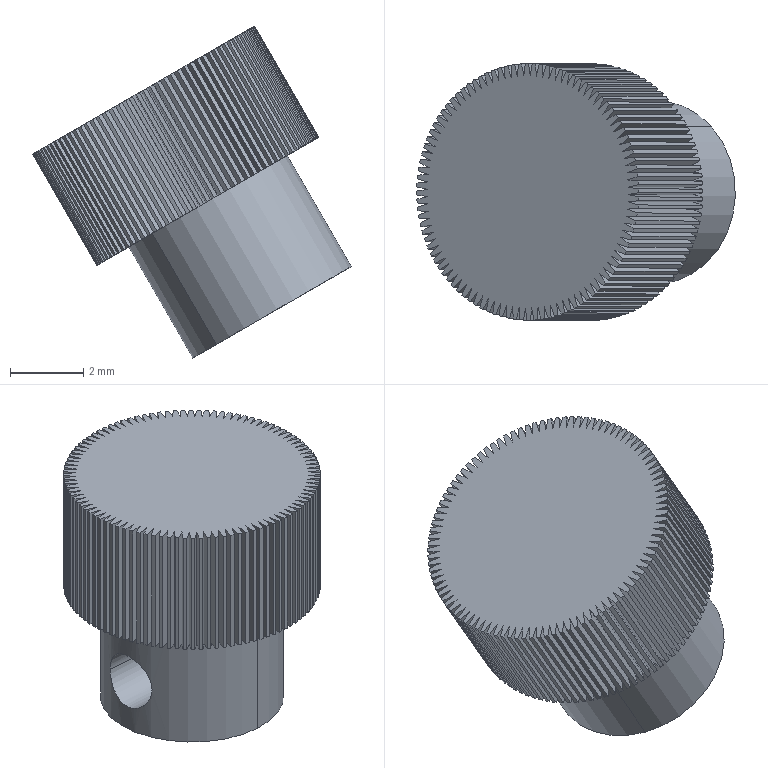Component | SolidWorks | SliderNut2-2 | 1 solid | 310 faces | box 8.7 x 7 x 9.06 mm | volume 183 mm3 | plane 204 | cylinder 106 | commonest cylinder face diameters 7 x100 1.6 x2 2 x2 5 x2
build123d program:
from build123d import *

# Parameters (mm, degrees)
SKETCH2_R               = 1
CUT_EXTRUDE1_DEPTH      = 3.5
CUT_EXTRUDE2_REACH      = 9.778
CUT_EXTRUDE2_END_RADIUS = 1
SKETCH3_R               = 0.8
CUT_EXTRUDE3_DEPTH      = 3.5


with BuildPart() as part:
    # Sketch1 → Revolve1 (revolve)
    with BuildSketch(Plane.XY, mode=Mode.PRIVATE) as revolve1_sk:
        Polygon((-3.5, 0), (3.5, 0), (3.5, 2.5), (0, 2.5), (0, 3.5), (-3.5, 3.5), align=None)
    revolve(revolve1_sk.sketch.rotate(Axis((-3.5, 0, 0), (1, 0, 0)), 90), axis=Axis((-3.5, 0, 0), (1, 0, 0)))

    # Sketch2 → Cut-Extrude1 (cut)
    with BuildSketch(Plane(origin=(3.5, 0, 0), x_dir=(0, 0, -1), z_dir=(1, 0, 0))):
        Circle(SKETCH2_R)
    extrude(amount=-CUT_EXTRUDE1_DEPTH, mode=Mode.SUBTRACT)

    # Cut-Extrude2: up to this cylinder (the profile starts outside it)
    cut_extrude2_end = Plane(origin=(2, 0, 0), z_dir=(1, 0, 0)) * Cylinder(CUT_EXTRUDE2_END_RADIUS, 22.556, mode=Mode.PRIVATE)
    # Sketch3 → Cut-Extrude2 (cut, up to the surface)
    with BuildSketch(Plane(origin=(0, 2.5, 0), x_dir=(1, 0, 0), z_dir=(0, 1, 0)), mode=Mode.PRIVATE) as cut_extrude2_sk1:
        with Locations(Location((2, 0, 0), (0, 0, 270))):
            Circle(SKETCH3_R)
    cut_extrude2_tool1 = extrude(cut_extrude2_sk1.sketch, amount=-CUT_EXTRUDE2_REACH, mode=Mode.PRIVATE) - cut_extrude2_end
    add(cut_extrude2_tool1.solids().sort_by_distance((2, 2.5, 0))[0], mode=Mode.SUBTRACT)

    # Sketch4 → Cut-Extrude3 (cut)
    with BuildSketch(Plane.ZY.offset(3.5)):
        Polygon((-0.1165, 3.83), (0, 3.17), (0.1165, 3.83), align=None)
        Polygon((0.1242, 3.83), (0.3567, 3.815), (0.1991, 3.164), align=None)
        Polygon((0.3644, 3.814), (0.5956, 3.785), (0.3973, 3.145), align=None)
        Polygon((0.6032, 3.784), (0.8321, 3.74), (0.594, 3.114), align=None)
        Polygon((0.8396, 3.739), (1.065, 3.681), (0.7884, 3.07), align=None)
        Polygon((1.073, 3.678), (1.294, 3.606), (0.9796, 3.015), align=None)
        Polygon((1.302, 3.604), (1.518, 3.518), (1.167, 2.947), align=None)
        Polygon((1.525, 3.515), (1.736, 3.416), (1.35, 2.868), align=None)
        Polygon((1.743, 3.412), (1.947, 3.3), (1.527, 2.778), align=None)
        Polygon((1.954, 3.296), (2.151, 3.171), (1.699, 2.677), align=None)
        Polygon((2.157, 3.167), (2.345, 3.03), (1.863, 2.565), align=None)
        Polygon((2.352, 3.025), (2.531, 2.877), (2.021, 2.443), align=None)
        Polygon((2.537, 2.872), (2.707, 2.712), (2.17, 2.311), align=None)
        Polygon((2.712, 2.707), (2.872, 2.537), (2.311, 2.17), align=None)
        Polygon((2.877, 2.531), (3.025, 2.352), (2.443, 2.021), align=None)
        Polygon((3.03, 2.345), (3.167, 2.157), (2.565, 1.863), align=None)
        Polygon((3.171, 2.151), (3.296, 1.954), (2.677, 1.699), align=None)
        Polygon((3.3, 1.947), (3.412, 1.743), (2.778, 1.527), align=None)
        Polygon((3.416, 1.736), (3.515, 1.525), (2.868, 1.35), align=None)
        Polygon((3.518, 1.518), (3.604, 1.302), (2.947, 1.167), align=None)
        Polygon((3.606, 1.294), (3.678, 1.073), (3.015, 0.9796), align=None)
        Polygon((3.681, 1.065), (3.739, 0.8396), (3.07, 0.7884), align=None)
        Polygon((3.74, 0.8321), (3.784, 0.6032), (3.114, 0.594), align=None)
        Polygon((3.785, 0.5956), (3.814, 0.3644), (3.145, 0.3973), align=None)
        Polygon((3.815, 0.3567), (3.83, 0.1242), (3.164, 0.1991), align=None)
        Polygon((3.83, 0.1165), (3.83, -0.1165), (3.17, 0), align=None)
        Polygon((3.83, -0.1242), (3.815, -0.3567), (3.164, -0.1991), align=None)
        Polygon((3.814, -0.3644), (3.785, -0.5956), (3.145, -0.3973), align=None)
        Polygon((3.784, -0.6032), (3.74, -0.8321), (3.114, -0.594), align=None)
        Polygon((3.739, -0.8396), (3.681, -1.065), (3.07, -0.7884), align=None)
        Polygon((3.678, -1.073), (3.606, -1.294), (3.015, -0.9796), align=None)
        Polygon((3.604, -1.302), (3.518, -1.518), (2.947, -1.167), align=None)
        Polygon((3.515, -1.525), (3.416, -1.736), (2.868, -1.35), align=None)
        Polygon((3.412, -1.743), (3.3, -1.947), (2.778, -1.527), align=None)
        Polygon((3.296, -1.954), (3.171, -2.151), (2.677, -1.699), align=None)
        Polygon((3.167, -2.157), (3.03, -2.345), (2.565, -1.863), align=None)
        Polygon((3.025, -2.352), (2.877, -2.531), (2.443, -2.021), align=None)
        Polygon((2.872, -2.537), (2.712, -2.707), (2.311, -2.17), align=None)
        Polygon((2.707, -2.712), (2.537, -2.872), (2.17, -2.311), align=None)
        Polygon((2.531, -2.877), (2.352, -3.025), (2.021, -2.443), align=None)
        Polygon((2.345, -3.03), (2.157, -3.167), (1.863, -2.565), align=None)
        Polygon((2.151, -3.171), (1.954, -3.296), (1.699, -2.677), align=None)
        Polygon((1.947, -3.3), (1.743, -3.412), (1.527, -2.778), align=None)
        Polygon((1.736, -3.416), (1.525, -3.515), (1.35, -2.868), align=None)
        Polygon((1.518, -3.518), (1.302, -3.604), (1.167, -2.947), align=None)
        Polygon((1.294, -3.606), (1.073, -3.678), (0.9796, -3.015), align=None)
        Polygon((1.065, -3.681), (0.8396, -3.739), (0.7884, -3.07), align=None)
        Polygon((0.8321, -3.74), (0.6032, -3.784), (0.594, -3.114), align=None)
        Polygon((0.5956, -3.785), (0.3644, -3.814), (0.3973, -3.145), align=None)
        Polygon((0.3567, -3.815), (0.1242, -3.83), (0.1991, -3.164), align=None)
        Polygon((0.1165, -3.83), (-0.1165, -3.83), (0, -3.17), align=None)
        Polygon((-0.1242, -3.83), (-0.3567, -3.815), (-0.1991, -3.164), align=None)
        Polygon((-0.3644, -3.814), (-0.5956, -3.785), (-0.3973, -3.145), align=None)
        Polygon((-0.6032, -3.784), (-0.8321, -3.74), (-0.594, -3.114), align=None)
        Polygon((-0.8396, -3.739), (-1.065, -3.681), (-0.7884, -3.07), align=None)
        Polygon((-1.073, -3.678), (-1.294, -3.606), (-0.9796, -3.015), align=None)
        Polygon((-1.302, -3.604), (-1.518, -3.518), (-1.167, -2.947), align=None)
        Polygon((-1.525, -3.515), (-1.736, -3.416), (-1.35, -2.868), align=None)
        Polygon((-1.743, -3.412), (-1.947, -3.3), (-1.527, -2.778), align=None)
        Polygon((-1.954, -3.296), (-2.151, -3.171), (-1.699, -2.677), align=None)
        Polygon((-2.157, -3.167), (-2.345, -3.03), (-1.863, -2.565), align=None)
        Polygon((-2.352, -3.025), (-2.531, -2.877), (-2.021, -2.443), align=None)
        Polygon((-2.537, -2.872), (-2.707, -2.712), (-2.17, -2.311), align=None)
        Polygon((-2.712, -2.707), (-2.872, -2.537), (-2.311, -2.17), align=None)
        Polygon((-2.877, -2.531), (-3.025, -2.352), (-2.443, -2.021), align=None)
        Polygon((-3.03, -2.345), (-3.167, -2.157), (-2.565, -1.863), align=None)
        Polygon((-3.171, -2.151), (-3.296, -1.954), (-2.677, -1.699), align=None)
        Polygon((-3.3, -1.947), (-3.412, -1.743), (-2.778, -1.527), align=None)
        Polygon((-3.416, -1.736), (-3.515, -1.525), (-2.868, -1.35), align=None)
        Polygon((-3.518, -1.518), (-3.604, -1.302), (-2.947, -1.167), align=None)
        Polygon((-3.606, -1.294), (-3.678, -1.073), (-3.015, -0.9796), align=None)
        Polygon((-3.681, -1.065), (-3.739, -0.8396), (-3.07, -0.7884), align=None)
        Polygon((-3.74, -0.8321), (-3.784, -0.6032), (-3.114, -0.594), align=None)
        Polygon((-3.785, -0.5956), (-3.814, -0.3644), (-3.145, -0.3973), align=None)
        Polygon((-3.815, -0.3567), (-3.83, -0.1242), (-3.164, -0.1991), align=None)
        Polygon((-3.83, -0.1165), (-3.83, 0.1165), (-3.17, 0), align=None)
        Polygon((-3.83, 0.1242), (-3.815, 0.3567), (-3.164, 0.1991), align=None)
        Polygon((-3.814, 0.3644), (-3.785, 0.5956), (-3.145, 0.3973), align=None)
        Polygon((-3.784, 0.6032), (-3.74, 0.8321), (-3.114, 0.594), align=None)
        Polygon((-3.739, 0.8396), (-3.681, 1.065), (-3.07, 0.7884), align=None)
        Polygon((-3.678, 1.073), (-3.606, 1.294), (-3.015, 0.9796), align=None)
        Polygon((-3.604, 1.302), (-3.518, 1.518), (-2.947, 1.167), align=None)
        Polygon((-3.515, 1.525), (-3.416, 1.736), (-2.868, 1.35), align=None)
        Polygon((-3.412, 1.743), (-3.3, 1.947), (-2.778, 1.527), align=None)
        Polygon((-3.296, 1.954), (-3.171, 2.151), (-2.677, 1.699), align=None)
        Polygon((-3.167, 2.157), (-3.03, 2.345), (-2.565, 1.863), align=None)
        Polygon((-3.025, 2.352), (-2.877, 2.531), (-2.443, 2.021), align=None)
        Polygon((-2.872, 2.537), (-2.712, 2.707), (-2.311, 2.17), align=None)
        Polygon((-2.707, 2.712), (-2.537, 2.872), (-2.17, 2.311), align=None)
        Polygon((-2.531, 2.877), (-2.352, 3.025), (-2.021, 2.443), align=None)
        Polygon((-2.345, 3.03), (-2.157, 3.167), (-1.863, 2.565), align=None)
        Polygon((-2.151, 3.171), (-1.954, 3.296), (-1.699, 2.677), align=None)
        Polygon((-1.947, 3.3), (-1.743, 3.412), (-1.527, 2.778), align=None)
        Polygon((-1.736, 3.416), (-1.525, 3.515), (-1.35, 2.868), align=None)
        Polygon((-1.518, 3.518), (-1.302, 3.604), (-1.167, 2.947), align=None)
        Polygon((-1.294, 3.606), (-1.073, 3.678), (-0.9796, 3.015), align=None)
        Polygon((-1.065, 3.681), (-0.8396, 3.739), (-0.7884, 3.07), align=None)
        Polygon((-0.8321, 3.74), (-0.6032, 3.784), (-0.594, 3.114), align=None)
        Polygon((-0.5956, 3.785), (-0.3644, 3.814), (-0.3973, 3.145), align=None)
        Polygon((-0.3567, 3.815), (-0.1242, 3.83), (-0.1991, 3.164), align=None)
    extrude(amount=-CUT_EXTRUDE3_DEPTH, mode=Mode.SUBTRACT)


solid = part.part

# Placed as in the assembly
solid = solid.moved(Location((-78.941, 33.561, 139.238), (-63.795, 37.411, 50.988)))